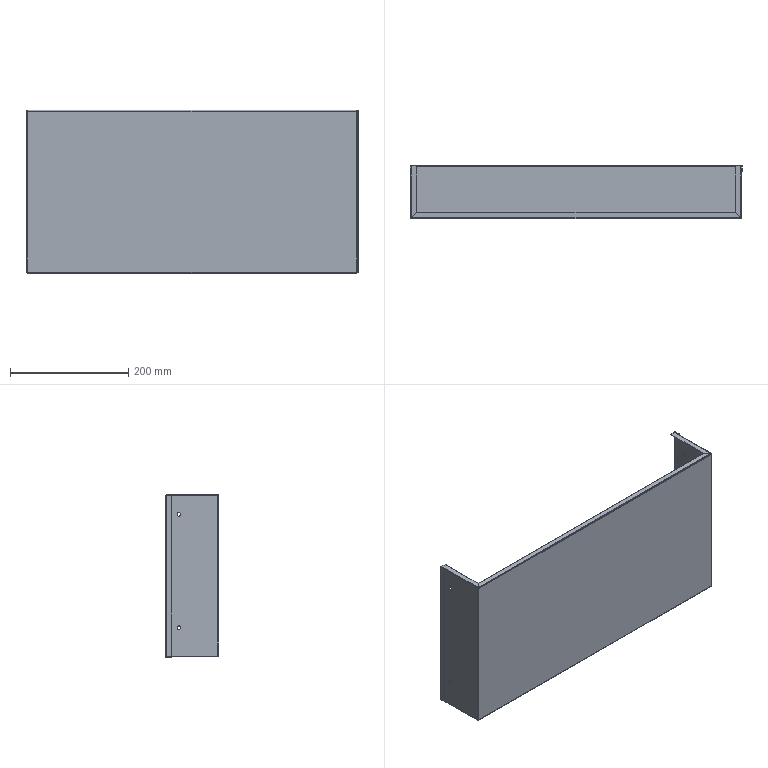Component | SolidWorks | PC-CAJ-P09-1_PC-CAJ-P15-1_PM-CAJ-P53-1 | 1 solid | 95 faces | volume 268197 mm3 | plane 62 | cylinder 29 | spline 4 | commonest cylinder face diameters 6 x8 1 x6 3 x6 2.2 x5 0.2 x4 | material Plain Carbon Steel